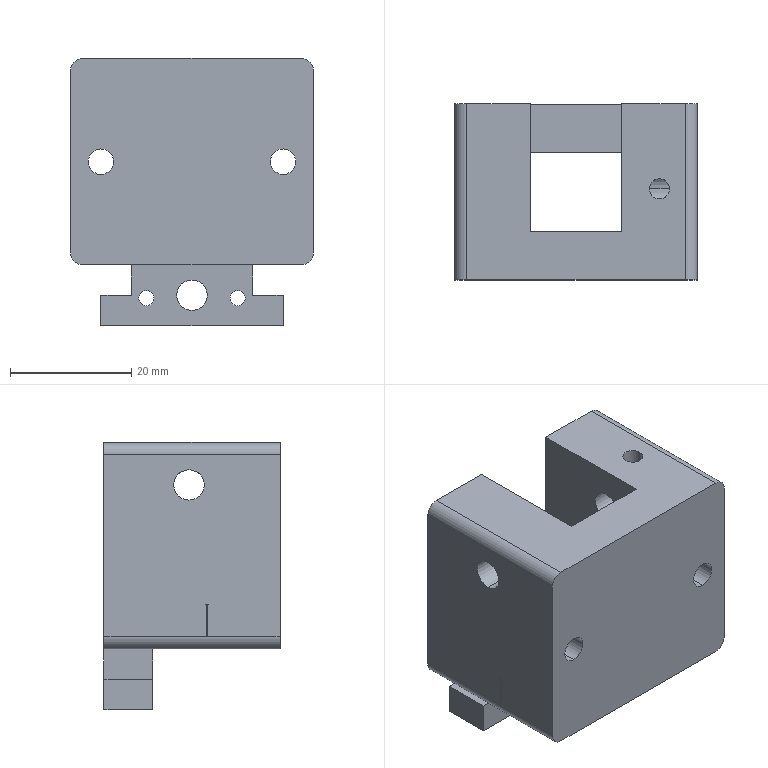Component | SolidWorks | 18ZTJ-NVT-01-005-1 | 1 solid | 74 faces | box 40 x 29 x 44 mm | volume 28872 mm3 | plane 34 | cylinder 24 | spline 16 | commonest cylinder face diameters 4 x6 5 x6 2.5 x4 4.2 x4 3.3 x2 5.8 x2 | material #45